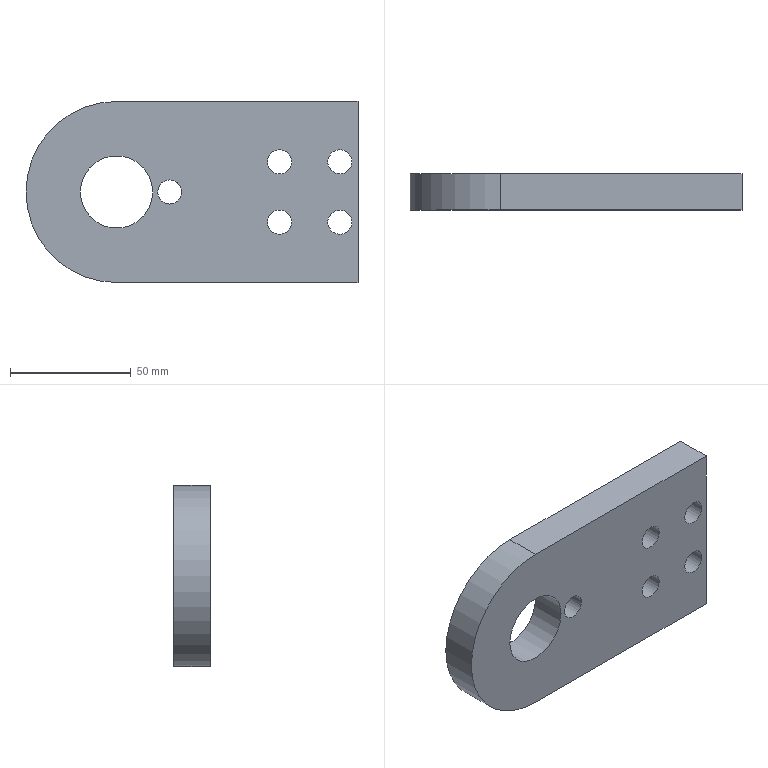Component | NX | DRILL_JIG_BUSH | 1 solid | 12 faces | box 137.5 x 15 x 75 mm | volume 129141 mm3 | cylinder 7 | plane 5 | commonest cylinder face diameters 10 x5 75 x1 30 x1
STEP:
#1=CARTESIAN_POINT('',(0.,0.,0.));
#2=DIRECTION('',(0.,0.,1.));
#3=DIRECTION('',(1.,0.,0.));
#4=AXIS2_PLACEMENT_3D('',#1,#2,#3);
#5=CARTESIAN_POINT('',(-28.675,85.796,25.));
#6=VERTEX_POINT('',#5);
#7=CARTESIAN_POINT('',(-28.675,85.796,100.));
#8=VERTEX_POINT('',#7);
#9=CARTESIAN_POINT('',(-28.675,85.796,62.5));
#10=DIRECTION('',(0.,1.,0.));
#11=DIRECTION('',(0.,0.,1.));
#12=AXIS2_PLACEMENT_3D('',#9,#10,#11);
#13=CIRCLE('',#12,37.5);
#14=CARTESIAN_POINT('',(-28.675,100.796,62.5));
#15=DIRECTION('',(0.,-1.,0.));
#16=DIRECTION('',(0.,0.,-1.));
#17=AXIS2_PLACEMENT_3D('',#14,#15,#16);
#18=CYLINDRICAL_SURFACE('',#17,37.5);
#19=CARTESIAN_POINT('',(9.425,15.));
#20=DIRECTION('',(-1.,0.));
#21=VECTOR('',#20,1.);
#22=LINE('',#19,#21);
#23=(GEOMETRIC_REPRESENTATION_CONTEXT(2)PARAMETRIC_REPRESENTATION_CONTEXT()REPRESENTATION_CONTEXT('',''));
#24=DEFINITIONAL_REPRESENTATION('',(#22),#23);
#25=PCURVE('',#18,#24);
#26=CARTESIAN_POINT('',(-28.675,85.796,62.5));
#27=DIRECTION('',(0.,1.,0.));
#28=DIRECTION('',(0.,0.,1.));
#29=AXIS2_PLACEMENT_3D('',#26,#27,#28);
#30=PLANE('',#29);
#31=CARTESIAN_POINT('',(0.,0.));
#32=DIRECTION('',(1.,0.));
#33=AXIS2_PLACEMENT_2D('',#31,#32);
#34=CIRCLE('',#33,37.5);
#35=(GEOMETRIC_REPRESENTATION_CONTEXT(2)PARAMETRIC_REPRESENTATION_CONTEXT()REPRESENTATION_CONTEXT('',''));
#36=DEFINITIONAL_REPRESENTATION('',(#34),#35);
#37=PCURVE('',#30,#36);
#38=SURFACE_CURVE('',#13,(#25,#37),.PCURVE_S1.);
#39=EDGE_CURVE('',#6,#8,#38,.T.);
#40=ORIENTED_EDGE('',*,*,#39,.T.);
#41=CARTESIAN_POINT('',(-28.675,100.796,100.));
#42=VERTEX_POINT('',#41);
#43=CARTESIAN_POINT('',(-28.675,93.296,100.));
#44=DIRECTION('',(0.,-1.,0.));
#45=VECTOR('',#44,1.);
#46=LINE('',#43,#45);
#47=CARTESIAN_POINT('',(3.142,7.5));
#48=DIRECTION('',(0.,1.));
#49=VECTOR('',#48,1.);
#50=LINE('',#47,#49);
#51=(GEOMETRIC_REPRESENTATION_CONTEXT(2)PARAMETRIC_REPRESENTATION_CONTEXT()REPRESENTATION_CONTEXT('',''));
#52=DEFINITIONAL_REPRESENTATION('',(#50),#51);
#53=PCURVE('',#18,#52);
#54=CARTESIAN_POINT('',(-28.675,100.796,100.));
#55=DIRECTION('',(0.,0.,-1.));
#56=DIRECTION('',(-1.,0.,0.));
#57=AXIS2_PLACEMENT_3D('',#54,#55,#56);
#58=PLANE('',#57);
#59=CARTESIAN_POINT('',(0.,-7.5));
#60=DIRECTION('',(0.,-1.));
#61=VECTOR('',#60,1.);
#62=LINE('',#59,#61);
#63=(GEOMETRIC_REPRESENTATION_CONTEXT(2)PARAMETRIC_REPRESENTATION_CONTEXT()REPRESENTATION_CONTEXT('',''));
#64=DEFINITIONAL_REPRESENTATION('',(#62),#63);
#65=PCURVE('',#58,#64);
#66=SURFACE_CURVE('',#46,(#53,#65),.PCURVE_S1.);
#67=EDGE_CURVE('',#42,#8,#66,.T.);
#68=ORIENTED_EDGE('',*,*,#67,.F.);
#69=CARTESIAN_POINT('',(-28.675,100.796,25.));
#70=VERTEX_POINT('',#69);
#71=CARTESIAN_POINT('',(-28.675,100.796,62.5));
#72=DIRECTION('',(0.,1.,0.));
#73=DIRECTION('',(0.,0.,1.));
#74=AXIS2_PLACEMENT_3D('',#71,#72,#73);
#75=CIRCLE('',#74,37.5);
#76=CARTESIAN_POINT('',(9.425,0.));
#77=DIRECTION('',(-1.,0.));
#78=VECTOR('',#77,1.);
#79=LINE('',#76,#78);
#80=(GEOMETRIC_REPRESENTATION_CONTEXT(2)PARAMETRIC_REPRESENTATION_CONTEXT()REPRESENTATION_CONTEXT('',''));
#81=DEFINITIONAL_REPRESENTATION('',(#79),#80);
#82=PCURVE('',#18,#81);
#83=CARTESIAN_POINT('',(-28.675,100.796,62.5));
#84=DIRECTION('',(0.,1.,0.));
#85=DIRECTION('',(0.,0.,1.));
#86=AXIS2_PLACEMENT_3D('',#83,#84,#85);
#87=PLANE('',#86);
#88=CARTESIAN_POINT('',(0.,0.));
#89=DIRECTION('',(1.,0.));
#90=AXIS2_PLACEMENT_2D('',#88,#89);
#91=CIRCLE('',#90,37.5);
#92=(GEOMETRIC_REPRESENTATION_CONTEXT(2)PARAMETRIC_REPRESENTATION_CONTEXT()REPRESENTATION_CONTEXT('',''));
#93=DEFINITIONAL_REPRESENTATION('',(#91),#92);
#94=PCURVE('',#87,#93);
#95=SURFACE_CURVE('',#75,(#82,#94),.PCURVE_S1.);
#96=EDGE_CURVE('',#70,#42,#95,.T.);
#97=ORIENTED_EDGE('',*,*,#96,.F.);
#98=CARTESIAN_POINT('',(-28.675,93.296,25.));
#99=DIRECTION('',(0.,-1.,0.));
#100=VECTOR('',#99,1.);
#101=LINE('',#98,#100);
#102=CARTESIAN_POINT('',(6.283,7.5));
#103=DIRECTION('',(0.,1.));
#104=VECTOR('',#103,1.);
#105=LINE('',#102,#104);
#106=(GEOMETRIC_REPRESENTATION_CONTEXT(2)PARAMETRIC_REPRESENTATION_CONTEXT()REPRESENTATION_CONTEXT('',''));
#107=DEFINITIONAL_REPRESENTATION('',(#105),#106);
#108=PCURVE('',#18,#107);
#109=CARTESIAN_POINT('',(71.325,100.796,25.));
#110=DIRECTION('',(0.,0.,1.));
#111=DIRECTION('',(1.,0.,0.));
#112=AXIS2_PLACEMENT_3D('',#109,#110,#111);
#113=PLANE('',#112);
#114=CARTESIAN_POINT('',(-100.,-7.5));
#115=DIRECTION('',(0.,-1.));
#116=VECTOR('',#115,1.);
#117=LINE('',#114,#116);
#118=(GEOMETRIC_REPRESENTATION_CONTEXT(2)PARAMETRIC_REPRESENTATION_CONTEXT()REPRESENTATION_CONTEXT('',''));
#119=DEFINITIONAL_REPRESENTATION('',(#117),#118);
#120=PCURVE('',#113,#119);
#121=SURFACE_CURVE('',#101,(#108,#120),.PCURVE_S1.);
#122=EDGE_CURVE('',#70,#6,#121,.T.);
#123=ORIENTED_EDGE('',*,*,#122,.T.);
#124=EDGE_LOOP('',(#40,#68,#97,#123));
#125=FACE_BOUND('',#124,.T.);
#126=ADVANCED_FACE('',(#125),#18,.T.);
#127=CARTESIAN_POINT('',(71.325,85.796,100.));
#128=VERTEX_POINT('',#127);
#129=CARTESIAN_POINT('',(-28.675,85.796,100.));
#130=DIRECTION('',(1.,0.,0.));
#131=VECTOR('',#130,1.);
#132=LINE('',#129,#131);
#133=CARTESIAN_POINT('',(0.,-15.));
#134=DIRECTION('',(-1.,0.));
#135=VECTOR('',#134,1.);
#136=LINE('',#133,#135);
#137=(GEOMETRIC_REPRESENTATION_CONTEXT(2)PARAMETRIC_REPRESENTATION_CONTEXT()REPRESENTATION_CONTEXT('',''));
#138=DEFINITIONAL_REPRESENTATION('',(#136),#137);
#139=PCURVE('',#58,#138);
#140=CARTESIAN_POINT('',(37.5,0.));
#141=DIRECTION('',(0.,1.));
#142=VECTOR('',#141,1.);
#143=LINE('',#140,#142);
#144=(GEOMETRIC_REPRESENTATION_CONTEXT(2)PARAMETRIC_REPRESENTATION_CONTEXT()REPRESENTATION_CONTEXT('',''));
#145=DEFINITIONAL_REPRESENTATION('',(#143),#144);
#146=PCURVE('',#30,#145);
#147=SURFACE_CURVE('',#132,(#139,#146),.PCURVE_S1.);
#148=EDGE_CURVE('',#8,#128,#147,.T.);
#149=ORIENTED_EDGE('',*,*,#148,.T.);
#150=CARTESIAN_POINT('',(71.325,100.796,100.));
#151=VERTEX_POINT('',#150);
#152=CARTESIAN_POINT('',(71.325,100.796,100.));
#153=DIRECTION('',(0.,-1.,0.));
#154=VECTOR('',#153,1.);
#155=LINE('',#152,#154);
#156=CARTESIAN_POINT('',(-100.,0.));
#157=DIRECTION('',(0.,-1.));
#158=VECTOR('',#157,1.);
#159=LINE('',#156,#158);
#160=(GEOMETRIC_REPRESENTATION_CONTEXT(2)PARAMETRIC_REPRESENTATION_CONTEXT()REPRESENTATION_CONTEXT('',''));
#161=DEFINITIONAL_REPRESENTATION('',(#159),#160);
#162=PCURVE('',#58,#161);
#163=CARTESIAN_POINT('',(71.325,100.796,112.5));
#164=DIRECTION('',(-1.,0.,-0.));
#165=DIRECTION('',(-0.,0.,1.));
#166=AXIS2_PLACEMENT_3D('',#163,#164,#165);
#167=PLANE('',#166);
#168=CARTESIAN_POINT('',(-12.5,0.));
#169=DIRECTION('',(0.,-1.));
#170=VECTOR('',#169,1.);
#171=LINE('',#168,#170);
#172=(GEOMETRIC_REPRESENTATION_CONTEXT(2)PARAMETRIC_REPRESENTATION_CONTEXT()REPRESENTATION_CONTEXT('',''));
#173=DEFINITIONAL_REPRESENTATION('',(#171),#172);
#174=PCURVE('',#167,#173);
#175=SURFACE_CURVE('',#155,(#162,#174),.PCURVE_S1.);
#176=EDGE_CURVE('',#151,#128,#175,.T.);
#177=ORIENTED_EDGE('',*,*,#176,.F.);
#178=CARTESIAN_POINT('',(-28.675,100.796,100.));
#179=DIRECTION('',(1.,0.,0.));
#180=VECTOR('',#179,1.);
#181=LINE('',#178,#180);
#182=CARTESIAN_POINT('',(0.,0.));
#183=DIRECTION('',(-1.,0.));
#184=VECTOR('',#183,1.);
#185=LINE('',#182,#184);
#186=(GEOMETRIC_REPRESENTATION_CONTEXT(2)PARAMETRIC_REPRESENTATION_CONTEXT()REPRESENTATION_CONTEXT('',''));
#187=DEFINITIONAL_REPRESENTATION('',(#185),#186);
#188=PCURVE('',#58,#187);
#189=CARTESIAN_POINT('',(37.5,0.));
#190=DIRECTION('',(0.,1.));
#191=VECTOR('',#190,1.);
#192=LINE('',#189,#191);
#193=(GEOMETRIC_REPRESENTATION_CONTEXT(2)PARAMETRIC_REPRESENTATION_CONTEXT()REPRESENTATION_CONTEXT('',''));
#194=DEFINITIONAL_REPRESENTATION('',(#192),#193);
#195=PCURVE('',#87,#194);
#196=SURFACE_CURVE('',#181,(#188,#195),.PCURVE_S1.);
#197=EDGE_CURVE('',#42,#151,#196,.T.);
#198=ORIENTED_EDGE('',*,*,#197,.F.);
#199=ORIENTED_EDGE('',*,*,#67,.T.);
#200=EDGE_LOOP('',(#149,#177,#198,#199));
#201=FACE_BOUND('',#200,.T.);
#202=ADVANCED_FACE('',(#201),#58,.F.);
#203=CARTESIAN_POINT('',(71.325,85.796,25.));
#204=VERTEX_POINT('',#203);
#205=CARTESIAN_POINT('',(71.325,85.796,112.5));
#206=DIRECTION('',(0.,0.,-1.));
#207=VECTOR('',#206,1.);
#208=LINE('',#205,#207);
#209=CARTESIAN_POINT('',(0.,-15.));
#210=DIRECTION('',(-1.,0.));
#211=VECTOR('',#210,1.);
#212=LINE('',#209,#211);
#213=(GEOMETRIC_REPRESENTATION_CONTEXT(2)PARAMETRIC_REPRESENTATION_CONTEXT()REPRESENTATION_CONTEXT('',''));
#214=DEFINITIONAL_REPRESENTATION('',(#212),#213);
#215=PCURVE('',#167,#214);
#216=CARTESIAN_POINT('',(50.,100.));
#217=DIRECTION('',(-1.,0.));
#218=VECTOR('',#217,1.);
#219=LINE('',#216,#218);
#220=(GEOMETRIC_REPRESENTATION_CONTEXT(2)PARAMETRIC_REPRESENTATION_CONTEXT()REPRESENTATION_CONTEXT('',''));
#221=DEFINITIONAL_REPRESENTATION('',(#219),#220);
#222=PCURVE('',#30,#221);
#223=SURFACE_CURVE('',#208,(#215,#222),.PCURVE_S1.);
#224=EDGE_CURVE('',#128,#204,#223,.T.);
#225=ORIENTED_EDGE('',*,*,#224,.T.);
#226=CARTESIAN_POINT('',(71.325,100.796,25.));
#227=VERTEX_POINT('',#226);
#228=CARTESIAN_POINT('',(71.325,100.796,25.));
#229=DIRECTION('',(0.,-1.,0.));
#230=VECTOR('',#229,1.);
#231=LINE('',#228,#230);
#232=CARTESIAN_POINT('',(-87.5,0.));
#233=DIRECTION('',(0.,-1.));
#234=VECTOR('',#233,1.);
#235=LINE('',#232,#234);
#236=(GEOMETRIC_REPRESENTATION_CONTEXT(2)PARAMETRIC_REPRESENTATION_CONTEXT()REPRESENTATION_CONTEXT('',''));
#237=DEFINITIONAL_REPRESENTATION('',(#235),#236);
#238=PCURVE('',#167,#237);
#239=CARTESIAN_POINT('',(0.,0.));
#240=DIRECTION('',(0.,-1.));
#241=VECTOR('',#240,1.);
#242=LINE('',#239,#241);
#243=(GEOMETRIC_REPRESENTATION_CONTEXT(2)PARAMETRIC_REPRESENTATION_CONTEXT()REPRESENTATION_CONTEXT('',''));
#244=DEFINITIONAL_REPRESENTATION('',(#242),#243);
#245=PCURVE('',#113,#244);
#246=SURFACE_CURVE('',#231,(#238,#245),.PCURVE_S1.);
#247=EDGE_CURVE('',#227,#204,#246,.T.);
#248=ORIENTED_EDGE('',*,*,#247,.F.);
#249=CARTESIAN_POINT('',(71.325,100.796,112.5));
#250=DIRECTION('',(0.,0.,-1.));
#251=VECTOR('',#250,1.);
#252=LINE('',#249,#251);
#253=CARTESIAN_POINT('',(0.,0.));
#254=DIRECTION('',(-1.,0.));
#255=VECTOR('',#254,1.);
#256=LINE('',#253,#255);
#257=(GEOMETRIC_REPRESENTATION_CONTEXT(2)PARAMETRIC_REPRESENTATION_CONTEXT()REPRESENTATION_CONTEXT('',''));
#258=DEFINITIONAL_REPRESENTATION('',(#256),#257);
#259=PCURVE('',#167,#258);
#260=CARTESIAN_POINT('',(50.,100.));
#261=DIRECTION('',(-1.,0.));
#262=VECTOR('',#261,1.);
#263=LINE('',#260,#262);
#264=(GEOMETRIC_REPRESENTATION_CONTEXT(2)PARAMETRIC_REPRESENTATION_CONTEXT()REPRESENTATION_CONTEXT('',''));
#265=DEFINITIONAL_REPRESENTATION('',(#263),#264);
#266=PCURVE('',#87,#265);
#267=SURFACE_CURVE('',#252,(#259,#266),.PCURVE_S1.);
#268=EDGE_CURVE('',#151,#227,#267,.T.);
#269=ORIENTED_EDGE('',*,*,#268,.F.);
#270=ORIENTED_EDGE('',*,*,#176,.T.);
#271=EDGE_LOOP('',(#225,#248,#269,#270));
#272=FACE_BOUND('',#271,.T.);
#273=ADVANCED_FACE('',(#272),#167,.F.);
#274=CARTESIAN_POINT('',(58.825,100.796,50.));
#275=VERTEX_POINT('',#274);
#276=CARTESIAN_POINT('',(63.825,100.796,50.));
#277=DIRECTION('',(0.,1.,0.));
#278=DIRECTION('',(-1.,0.,0.));
#279=AXIS2_PLACEMENT_3D('',#276,#277,#278);
#280=CIRCLE('',#279,5.);
#281=CARTESIAN_POINT('',(63.825,100.796,50.));
#282=DIRECTION('',(0.,-1.,0.));
#283=DIRECTION('',(0.,0.,-1.));
#284=AXIS2_PLACEMENT_3D('',#281,#282,#283);
#285=CYLINDRICAL_SURFACE('',#284,5.);
#286=CARTESIAN_POINT('',(10.996,0.));
#287=DIRECTION('',(-1.,0.));
#288=VECTOR('',#287,1.);
#289=LINE('',#286,#288);
#290=(GEOMETRIC_REPRESENTATION_CONTEXT(2)PARAMETRIC_REPRESENTATION_CONTEXT()REPRESENTATION_CONTEXT('',''));
#291=DEFINITIONAL_REPRESENTATION('',(#289),#290);
#292=PCURVE('',#285,#291);
#293=CARTESIAN_POINT('',(-12.5,92.5));
#294=DIRECTION('',(0.,-1.));
#295=AXIS2_PLACEMENT_2D('',#293,#294);
#296=CIRCLE('',#295,5.);
#297=(GEOMETRIC_REPRESENTATION_CONTEXT(2)PARAMETRIC_REPRESENTATION_CONTEXT()REPRESENTATION_CONTEXT('',''));
#298=DEFINITIONAL_REPRESENTATION('',(#296),#297);
#299=PCURVE('',#87,#298);
#300=SURFACE_CURVE('',#280,(#292,#299),.PCURVE_S1.);
#301=EDGE_CURVE('',#275,#275,#300,.T.);
#302=ORIENTED_EDGE('',*,*,#301,.F.);
#303=CARTESIAN_POINT('',(58.825,85.796,50.));
#304=VERTEX_POINT('',#303);
#305=CARTESIAN_POINT('',(58.825,100.796,50.));
#306=CARTESIAN_POINT('',(58.825,85.796,50.));
#307=B_SPLINE_CURVE_WITH_KNOTS('',1,(#305,#306),.UNSPECIFIED.,.F.,.F.,(2,2),(0.,15.),.PIECEWISE_BEZIER_KNOTS.);
#308=CARTESIAN_POINT('',(10.996,0.));
#309=DIRECTION('',(0.,1.));
#310=VECTOR('',#309,1.);
#311=LINE('',#308,#310);
#312=(GEOMETRIC_REPRESENTATION_CONTEXT(2)PARAMETRIC_REPRESENTATION_CONTEXT()REPRESENTATION_CONTEXT('',''));
#313=DEFINITIONAL_REPRESENTATION('',(#311),#312);
#314=PCURVE('',#285,#313);
#315=CARTESIAN_POINT('',(4.712,0.));
#316=DIRECTION('',(0.,1.));
#317=VECTOR('',#316,1.);
#318=LINE('',#315,#317);
#319=(GEOMETRIC_REPRESENTATION_CONTEXT(2)PARAMETRIC_REPRESENTATION_CONTEXT()REPRESENTATION_CONTEXT('',''));
#320=DEFINITIONAL_REPRESENTATION('',(#318),#319);
#321=PCURVE('',#285,#320);
#322=SEAM_CURVE('',#307,(#314,#321),.PCURVE_S1.);
#323=EDGE_CURVE('',#275,#304,#322,.T.);
#324=ORIENTED_EDGE('',*,*,#323,.T.);
#325=CARTESIAN_POINT('',(63.825,85.796,50.));
#326=DIRECTION('',(0.,1.,0.));
#327=DIRECTION('',(-1.,0.,0.));
#328=AXIS2_PLACEMENT_3D('',#325,#326,#327);
#329=CIRCLE('',#328,5.);
#330=CARTESIAN_POINT('',(10.996,15.));
#331=DIRECTION('',(-1.,0.));
#332=VECTOR('',#331,1.);
#333=LINE('',#330,#332);
#334=(GEOMETRIC_REPRESENTATION_CONTEXT(2)PARAMETRIC_REPRESENTATION_CONTEXT()REPRESENTATION_CONTEXT('',''));
#335=DEFINITIONAL_REPRESENTATION('',(#333),#334);
#336=PCURVE('',#285,#335);
#337=CARTESIAN_POINT('',(-12.5,92.5));
#338=DIRECTION('',(0.,-1.));
#339=AXIS2_PLACEMENT_2D('',#337,#338);
#340=CIRCLE('',#339,5.);
#341=(GEOMETRIC_REPRESENTATION_CONTEXT(2)PARAMETRIC_REPRESENTATION_CONTEXT()REPRESENTATION_CONTEXT('',''));
#342=DEFINITIONAL_REPRESENTATION('',(#340),#341);
#343=PCURVE('',#30,#342);
#344=SURFACE_CURVE('',#329,(#336,#343),.PCURVE_S1.);
#345=EDGE_CURVE('',#304,#304,#344,.T.);
#346=ORIENTED_EDGE('',*,*,#345,.T.);
#347=ORIENTED_EDGE('',*,*,#323,.F.);
#348=EDGE_LOOP('',(#302,#324,#346,#347));
#349=FACE_BOUND('',#348,.F.);
#350=ADVANCED_FACE('',(#349),#285,.F.);
#351=CARTESIAN_POINT('',(33.825,100.796,75.));
#352=VERTEX_POINT('',#351);
#353=CARTESIAN_POINT('',(38.825,100.796,75.));
#354=DIRECTION('',(0.,1.,0.));
#355=DIRECTION('',(-1.,0.,0.));
#356=AXIS2_PLACEMENT_3D('',#353,#354,#355);
#357=CIRCLE('',#356,5.);
#358=CARTESIAN_POINT('',(38.825,100.796,75.));
#359=DIRECTION('',(0.,-1.,0.));
#360=DIRECTION('',(0.,0.,-1.));
#361=AXIS2_PLACEMENT_3D('',#358,#359,#360);
#362=CYLINDRICAL_SURFACE('',#361,5.);
#363=CARTESIAN_POINT('',(10.996,0.));
#364=DIRECTION('',(-1.,0.));
#365=VECTOR('',#364,1.);
#366=LINE('',#363,#365);
#367=(GEOMETRIC_REPRESENTATION_CONTEXT(2)PARAMETRIC_REPRESENTATION_CONTEXT()REPRESENTATION_CONTEXT('',''));
#368=DEFINITIONAL_REPRESENTATION('',(#366),#367);
#369=PCURVE('',#362,#368);
#370=CARTESIAN_POINT('',(12.5,67.5));
#371=DIRECTION('',(0.,-1.));
#372=AXIS2_PLACEMENT_2D('',#370,#371);
#373=CIRCLE('',#372,5.);
#374=(GEOMETRIC_REPRESENTATION_CONTEXT(2)PARAMETRIC_REPRESENTATION_CONTEXT()REPRESENTATION_CONTEXT('',''));
#375=DEFINITIONAL_REPRESENTATION('',(#373),#374);
#376=PCURVE('',#87,#375);
#377=SURFACE_CURVE('',#357,(#369,#376),.PCURVE_S1.);
#378=EDGE_CURVE('',#352,#352,#377,.T.);
#379=ORIENTED_EDGE('',*,*,#378,.F.);
#380=CARTESIAN_POINT('',(33.825,85.796,75.));
#381=VERTEX_POINT('',#380);
#382=CARTESIAN_POINT('',(33.825,100.796,75.));
#383=CARTESIAN_POINT('',(33.825,85.796,75.));
#384=B_SPLINE_CURVE_WITH_KNOTS('',1,(#382,#383),.UNSPECIFIED.,.F.,.F.,(2,2),(0.,15.),.PIECEWISE_BEZIER_KNOTS.);
#385=CARTESIAN_POINT('',(10.996,0.));
#386=DIRECTION('',(0.,1.));
#387=VECTOR('',#386,1.);
#388=LINE('',#385,#387);
#389=(GEOMETRIC_REPRESENTATION_CONTEXT(2)PARAMETRIC_REPRESENTATION_CONTEXT()REPRESENTATION_CONTEXT('',''));
#390=DEFINITIONAL_REPRESENTATION('',(#388),#389);
#391=PCURVE('',#362,#390);
#392=CARTESIAN_POINT('',(4.712,0.));
#393=DIRECTION('',(0.,1.));
#394=VECTOR('',#393,1.);
#395=LINE('',#392,#394);
#396=(GEOMETRIC_REPRESENTATION_CONTEXT(2)PARAMETRIC_REPRESENTATION_CONTEXT()REPRESENTATION_CONTEXT('',''));
#397=DEFINITIONAL_REPRESENTATION('',(#395),#396);
#398=PCURVE('',#362,#397);
#399=SEAM_CURVE('',#384,(#391,#398),.PCURVE_S1.);
#400=EDGE_CURVE('',#352,#381,#399,.T.);
#401=ORIENTED_EDGE('',*,*,#400,.T.);
#402=CARTESIAN_POINT('',(38.825,85.796,75.));
#403=DIRECTION('',(0.,1.,0.));
#404=DIRECTION('',(-1.,0.,0.));
#405=AXIS2_PLACEMENT_3D('',#402,#403,#404);
#406=CIRCLE('',#405,5.);
#407=CARTESIAN_POINT('',(10.996,15.));
#408=DIRECTION('',(-1.,0.));
#409=VECTOR('',#408,1.);
#410=LINE('',#407,#409);
#411=(GEOMETRIC_REPRESENTATION_CONTEXT(2)PARAMETRIC_REPRESENTATION_CONTEXT()REPRESENTATION_CONTEXT('',''));
#412=DEFINITIONAL_REPRESENTATION('',(#410),#411);
#413=PCURVE('',#362,#412);
#414=CARTESIAN_POINT('',(12.5,67.5));
#415=DIRECTION('',(0.,-1.));
#416=AXIS2_PLACEMENT_2D('',#414,#415);
#417=CIRCLE('',#416,5.);
#418=(GEOMETRIC_REPRESENTATION_CONTEXT(2)PARAMETRIC_REPRESENTATION_CONTEXT()REPRESENTATION_CONTEXT('',''));
#419=DEFINITIONAL_REPRESENTATION('',(#417),#418);
#420=PCURVE('',#30,#419);
#421=SURFACE_CURVE('',#406,(#413,#420),.PCURVE_S1.);
#422=EDGE_CURVE('',#381,#381,#421,.T.);
#423=ORIENTED_EDGE('',*,*,#422,.T.);
#424=ORIENTED_EDGE('',*,*,#400,.F.);
#425=EDGE_LOOP('',(#379,#401,#423,#424));
#426=FACE_BOUND('',#425,.F.);
#427=ADVANCED_FACE('',(#426),#362,.F.);
#428=CARTESIAN_POINT('',(33.825,100.796,50.));
#429=VERTEX_POINT('',#428);
#430=CARTESIAN_POINT('',(38.825,100.796,50.));
#431=DIRECTION('',(0.,1.,0.));
#432=DIRECTION('',(-1.,0.,0.));
#433=AXIS2_PLACEMENT_3D('',#430,#431,#432);
#434=CIRCLE('',#433,5.);
#435=CARTESIAN_POINT('',(38.825,100.796,50.));
#436=DIRECTION('',(0.,-1.,0.));
#437=DIRECTION('',(0.,0.,-1.));
#438=AXIS2_PLACEMENT_3D('',#435,#436,#437);
#439=CYLINDRICAL_SURFACE('',#438,5.);
#440=CARTESIAN_POINT('',(10.996,0.));
#441=DIRECTION('',(-1.,0.));
#442=VECTOR('',#441,1.);
#443=LINE('',#440,#442);
#444=(GEOMETRIC_REPRESENTATION_CONTEXT(2)PARAMETRIC_REPRESENTATION_CONTEXT()REPRESENTATION_CONTEXT('',''));
#445=DEFINITIONAL_REPRESENTATION('',(#443),#444);
#446=PCURVE('',#439,#445);
#447=CARTESIAN_POINT('',(-12.5,67.5));
#448=DIRECTION('',(0.,-1.));
#449=AXIS2_PLACEMENT_2D('',#447,#448);
#450=CIRCLE('',#449,5.);
#451=(GEOMETRIC_REPRESENTATION_CONTEXT(2)PARAMETRIC_REPRESENTATION_CONTEXT()REPRESENTATION_CONTEXT('',''));
#452=DEFINITIONAL_REPRESENTATION('',(#450),#451);
#453=PCURVE('',#87,#452);
#454=SURFACE_CURVE('',#434,(#446,#453),.PCURVE_S1.);
#455=EDGE_CURVE('',#429,#429,#454,.T.);
#456=ORIENTED_EDGE('',*,*,#455,.F.);
#457=CARTESIAN_POINT('',(33.825,85.796,50.));
#458=VERTEX_POINT('',#457);
#459=CARTESIAN_POINT('',(33.825,100.796,50.));
#460=CARTESIAN_POINT('',(33.825,85.796,50.));
#461=B_SPLINE_CURVE_WITH_KNOTS('',1,(#459,#460),.UNSPECIFIED.,.F.,.F.,(2,2),(0.,15.),.PIECEWISE_BEZIER_KNOTS.);
#462=CARTESIAN_POINT('',(10.996,0.));
#463=DIRECTION('',(0.,1.));
#464=VECTOR('',#463,1.);
#465=LINE('',#462,#464);
#466=(GEOMETRIC_REPRESENTATION_CONTEXT(2)PARAMETRIC_REPRESENTATION_CONTEXT()REPRESENTATION_CONTEXT('',''));
#467=DEFINITIONAL_REPRESENTATION('',(#465),#466);
#468=PCURVE('',#439,#467);
#469=CARTESIAN_POINT('',(4.712,0.));
#470=DIRECTION('',(0.,1.));
#471=VECTOR('',#470,1.);
#472=LINE('',#469,#471);
#473=(GEOMETRIC_REPRESENTATION_CONTEXT(2)PARAMETRIC_REPRESENTATION_CONTEXT()REPRESENTATION_CONTEXT('',''));
#474=DEFINITIONAL_REPRESENTATION('',(#472),#473);
#475=PCURVE('',#439,#474);
#476=SEAM_CURVE('',#461,(#468,#475),.PCURVE_S1.);
#477=EDGE_CURVE('',#429,#458,#476,.T.);
#478=ORIENTED_EDGE('',*,*,#477,.T.);
#479=CARTESIAN_POINT('',(38.825,85.796,50.));
#480=DIRECTION('',(0.,1.,0.));
#481=DIRECTION('',(-1.,0.,0.));
#482=AXIS2_PLACEMENT_3D('',#479,#480,#481);
#483=CIRCLE('',#482,5.);
#484=CARTESIAN_POINT('',(10.996,15.));
#485=DIRECTION('',(-1.,0.));
#486=VECTOR('',#485,1.);
#487=LINE('',#484,#486);
#488=(GEOMETRIC_REPRESENTATION_CONTEXT(2)PARAMETRIC_REPRESENTATION_CONTEXT()REPRESENTATION_CONTEXT('',''));
#489=DEFINITIONAL_REPRESENTATION('',(#487),#488);
#490=PCURVE('',#439,#489);
#491=CARTESIAN_POINT('',(-12.5,67.5));
#492=DIRECTION('',(0.,-1.));
#493=AXIS2_PLACEMENT_2D('',#491,#492);
#494=CIRCLE('',#493,5.);
#495=(GEOMETRIC_REPRESENTATION_CONTEXT(2)PARAMETRIC_REPRESENTATION_CONTEXT()REPRESENTATION_CONTEXT('',''));
#496=DEFINITIONAL_REPRESENTATION('',(#494),#495);
#497=PCURVE('',#30,#496);
#498=SURFACE_CURVE('',#483,(#490,#497),.PCURVE_S1.);
#499=EDGE_CURVE('',#458,#458,#498,.T.);
#500=ORIENTED_EDGE('',*,*,#499,.T.);
#501=ORIENTED_EDGE('',*,*,#477,.F.);
#502=EDGE_LOOP('',(#456,#478,#500,#501));
#503=FACE_BOUND('',#502,.F.);
#504=ADVANCED_FACE('',(#503),#439,.F.);
#505=CARTESIAN_POINT('',(-43.675,100.796,62.5));
#506=VERTEX_POINT('',#505);
#507=CARTESIAN_POINT('',(-28.675,100.796,62.5));
#508=DIRECTION('',(0.,1.,0.));
#509=DIRECTION('',(-1.,0.,0.));
#510=AXIS2_PLACEMENT_3D('',#507,#508,#509);
#511=CIRCLE('',#510,15.);
#512=CARTESIAN_POINT('',(-28.675,100.796,62.5));
#513=DIRECTION('',(0.,-1.,0.));
#514=DIRECTION('',(0.,0.,-1.));
#515=AXIS2_PLACEMENT_3D('',#512,#513,#514);
#516=CYLINDRICAL_SURFACE('',#515,15.);
#517=CARTESIAN_POINT('',(10.996,0.));
#518=DIRECTION('',(-1.,0.));
#519=VECTOR('',#518,1.);
#520=LINE('',#517,#519);
#521=(GEOMETRIC_REPRESENTATION_CONTEXT(2)PARAMETRIC_REPRESENTATION_CONTEXT()REPRESENTATION_CONTEXT('',''));
#522=DEFINITIONAL_REPRESENTATION('',(#520),#521);
#523=PCURVE('',#516,#522);
#524=CARTESIAN_POINT('',(0.,0.));
#525=DIRECTION('',(0.,-1.));
#526=AXIS2_PLACEMENT_2D('',#524,#525);
#527=CIRCLE('',#526,15.);
#528=(GEOMETRIC_REPRESENTATION_CONTEXT(2)PARAMETRIC_REPRESENTATION_CONTEXT()REPRESENTATION_CONTEXT('',''));
#529=DEFINITIONAL_REPRESENTATION('',(#527),#528);
#530=PCURVE('',#87,#529);
#531=SURFACE_CURVE('',#511,(#523,#530),.PCURVE_S1.);
#532=EDGE_CURVE('',#506,#506,#531,.T.);
#533=ORIENTED_EDGE('',*,*,#532,.F.);
#534=CARTESIAN_POINT('',(-43.675,85.796,62.5));
#535=VERTEX_POINT('',#534);
#536=CARTESIAN_POINT('',(-43.675,100.796,62.5));
#537=CARTESIAN_POINT('',(-43.675,85.796,62.5));
#538=B_SPLINE_CURVE_WITH_KNOTS('',1,(#536,#537),.UNSPECIFIED.,.F.,.F.,(2,2),(0.,15.),.PIECEWISE_BEZIER_KNOTS.);
#539=CARTESIAN_POINT('',(10.996,0.));
#540=DIRECTION('',(0.,1.));
#541=VECTOR('',#540,1.);
#542=LINE('',#539,#541);
#543=(GEOMETRIC_REPRESENTATION_CONTEXT(2)PARAMETRIC_REPRESENTATION_CONTEXT()REPRESENTATION_CONTEXT('',''));
#544=DEFINITIONAL_REPRESENTATION('',(#542),#543);
#545=PCURVE('',#516,#544);
#546=CARTESIAN_POINT('',(4.712,0.));
#547=DIRECTION('',(0.,1.));
#548=VECTOR('',#547,1.);
#549=LINE('',#546,#548);
#550=(GEOMETRIC_REPRESENTATION_CONTEXT(2)PARAMETRIC_REPRESENTATION_CONTEXT()REPRESENTATION_CONTEXT('',''));
#551=DEFINITIONAL_REPRESENTATION('',(#549),#550);
#552=PCURVE('',#516,#551);
#553=SEAM_CURVE('',#538,(#545,#552),.PCURVE_S1.);
#554=EDGE_CURVE('',#506,#535,#553,.T.);
#555=ORIENTED_EDGE('',*,*,#554,.T.);
#556=CARTESIAN_POINT('',(-28.675,85.796,62.5));
#557=DIRECTION('',(0.,1.,0.));
#558=DIRECTION('',(-1.,0.,0.));
#559=AXIS2_PLACEMENT_3D('',#556,#557,#558);
#560=CIRCLE('',#559,15.);
#561=CARTESIAN_POINT('',(10.996,15.));
#562=DIRECTION('',(-1.,0.));
#563=VECTOR('',#562,1.);
#564=LINE('',#561,#563);
#565=(GEOMETRIC_REPRESENTATION_CONTEXT(2)PARAMETRIC_REPRESENTATION_CONTEXT()REPRESENTATION_CONTEXT('',''));
#566=DEFINITIONAL_REPRESENTATION('',(#564),#565);
#567=PCURVE('',#516,#566);
#568=CARTESIAN_POINT('',(0.,0.));
#569=DIRECTION('',(0.,-1.));
#570=AXIS2_PLACEMENT_2D('',#568,#569);
#571=CIRCLE('',#570,15.);
#572=(GEOMETRIC_REPRESENTATION_CONTEXT(2)PARAMETRIC_REPRESENTATION_CONTEXT()REPRESENTATION_CONTEXT('',''));
#573=DEFINITIONAL_REPRESENTATION('',(#571),#572);
#574=PCURVE('',#30,#573);
#575=SURFACE_CURVE('',#560,(#567,#574),.PCURVE_S1.);
#576=EDGE_CURVE('',#535,#535,#575,.T.);
#577=ORIENTED_EDGE('',*,*,#576,.T.);
#578=ORIENTED_EDGE('',*,*,#554,.F.);
#579=EDGE_LOOP('',(#533,#555,#577,#578));
#580=FACE_BOUND('',#579,.F.);
#581=ADVANCED_FACE('',(#580),#516,.F.);
#582=CARTESIAN_POINT('',(71.325,85.796,25.));
#583=DIRECTION('',(-1.,0.,0.));
#584=VECTOR('',#583,1.);
#585=LINE('',#582,#584);
#586=CARTESIAN_POINT('',(0.,-15.));
#587=DIRECTION('',(-1.,0.));
#588=VECTOR('',#587,1.);
#589=LINE('',#586,#588);
#590=(GEOMETRIC_REPRESENTATION_CONTEXT(2)PARAMETRIC_REPRESENTATION_CONTEXT()REPRESENTATION_CONTEXT('',''));
#591=DEFINITIONAL_REPRESENTATION('',(#589),#590);
#592=PCURVE('',#113,#591);
#593=CARTESIAN_POINT('',(-37.5,100.));
#594=DIRECTION('',(0.,-1.));
#595=VECTOR('',#594,1.);
#596=LINE('',#593,#595);
#597=(GEOMETRIC_REPRESENTATION_CONTEXT(2)PARAMETRIC_REPRESENTATION_CONTEXT()REPRESENTATION_CONTEXT('',''));
#598=DEFINITIONAL_REPRESENTATION('',(#596),#597);
#599=PCURVE('',#30,#598);
#600=SURFACE_CURVE('',#585,(#592,#599),.PCURVE_S1.);
#601=EDGE_CURVE('',#204,#6,#600,.T.);
#602=ORIENTED_EDGE('',*,*,#601,.T.);
#603=ORIENTED_EDGE('',*,*,#122,.F.);
#604=CARTESIAN_POINT('',(71.325,100.796,25.));
#605=DIRECTION('',(-1.,0.,0.));
#606=VECTOR('',#605,1.);
#607=LINE('',#604,#606);
#608=CARTESIAN_POINT('',(0.,0.));
#609=DIRECTION('',(-1.,0.));
#610=VECTOR('',#609,1.);
#611=LINE('',#608,#610);
#612=(GEOMETRIC_REPRESENTATION_CONTEXT(2)PARAMETRIC_REPRESENTATION_CONTEXT()REPRESENTATION_CONTEXT('',''));
#613=DEFINITIONAL_REPRESENTATION('',(#611),#612);
#614=PCURVE('',#113,#613);
#615=CARTESIAN_POINT('',(-37.5,100.));
#616=DIRECTION('',(0.,-1.));
#617=VECTOR('',#616,1.);
#618=LINE('',#615,#617);
#619=(GEOMETRIC_REPRESENTATION_CONTEXT(2)PARAMETRIC_REPRESENTATION_CONTEXT()REPRESENTATION_CONTEXT('',''));
#620=DEFINITIONAL_REPRESENTATION('',(#618),#619);
#621=PCURVE('',#87,#620);
#622=SURFACE_CURVE('',#607,(#614,#621),.PCURVE_S1.);
#623=EDGE_CURVE('',#227,#70,#622,.T.);
#624=ORIENTED_EDGE('',*,*,#623,.F.);
#625=ORIENTED_EDGE('',*,*,#247,.T.);
#626=EDGE_LOOP('',(#602,#603,#624,#625));
#627=FACE_BOUND('',#626,.T.);
#628=ADVANCED_FACE('',(#627),#113,.F.);
#629=CARTESIAN_POINT('',(58.825,100.796,75.));
#630=VERTEX_POINT('',#629);
#631=CARTESIAN_POINT('',(63.825,100.796,75.));
#632=DIRECTION('',(0.,1.,0.));
#633=DIRECTION('',(-1.,0.,0.));
#634=AXIS2_PLACEMENT_3D('',#631,#632,#633);
#635=CIRCLE('',#634,5.);
#636=CARTESIAN_POINT('',(63.825,100.796,75.));
#637=DIRECTION('',(0.,-1.,0.));
#638=DIRECTION('',(0.,0.,-1.));
#639=AXIS2_PLACEMENT_3D('',#636,#637,#638);
#640=CYLINDRICAL_SURFACE('',#639,5.);
#641=CARTESIAN_POINT('',(10.996,0.));
#642=DIRECTION('',(-1.,0.));
#643=VECTOR('',#642,1.);
#644=LINE('',#641,#643);
#645=(GEOMETRIC_REPRESENTATION_CONTEXT(2)PARAMETRIC_REPRESENTATION_CONTEXT()REPRESENTATION_CONTEXT('',''));
#646=DEFINITIONAL_REPRESENTATION('',(#644),#645);
#647=PCURVE('',#640,#646);
#648=CARTESIAN_POINT('',(12.5,92.5));
#649=DIRECTION('',(0.,-1.));
#650=AXIS2_PLACEMENT_2D('',#648,#649);
#651=CIRCLE('',#650,5.);
#652=(GEOMETRIC_REPRESENTATION_CONTEXT(2)PARAMETRIC_REPRESENTATION_CONTEXT()REPRESENTATION_CONTEXT('',''));
#653=DEFINITIONAL_REPRESENTATION('',(#651),#652);
#654=PCURVE('',#87,#653);
#655=SURFACE_CURVE('',#635,(#647,#654),.PCURVE_S1.);
#656=EDGE_CURVE('',#630,#630,#655,.T.);
#657=ORIENTED_EDGE('',*,*,#656,.F.);
#658=CARTESIAN_POINT('',(58.825,85.796,75.));
#659=VERTEX_POINT('',#658);
#660=CARTESIAN_POINT('',(58.825,100.796,75.));
#661=CARTESIAN_POINT('',(58.825,85.796,75.));
#662=B_SPLINE_CURVE_WITH_KNOTS('',1,(#660,#661),.UNSPECIFIED.,.F.,.F.,(2,2),(0.,15.),.PIECEWISE_BEZIER_KNOTS.);
#663=CARTESIAN_POINT('',(10.996,0.));
#664=DIRECTION('',(0.,1.));
#665=VECTOR('',#664,1.);
#666=LINE('',#663,#665);
#667=(GEOMETRIC_REPRESENTATION_CONTEXT(2)PARAMETRIC_REPRESENTATION_CONTEXT()REPRESENTATION_CONTEXT('',''));
#668=DEFINITIONAL_REPRESENTATION('',(#666),#667);
#669=PCURVE('',#640,#668);
#670=CARTESIAN_POINT('',(4.712,0.));
#671=DIRECTION('',(0.,1.));
#672=VECTOR('',#671,1.);
#673=LINE('',#670,#672);
#674=(GEOMETRIC_REPRESENTATION_CONTEXT(2)PARAMETRIC_REPRESENTATION_CONTEXT()REPRESENTATION_CONTEXT('',''));
#675=DEFINITIONAL_REPRESENTATION('',(#673),#674);
#676=PCURVE('',#640,#675);
#677=SEAM_CURVE('',#662,(#669,#676),.PCURVE_S1.);
#678=EDGE_CURVE('',#630,#659,#677,.T.);
#679=ORIENTED_EDGE('',*,*,#678,.T.);
#680=CARTESIAN_POINT('',(63.825,85.796,75.));
#681=DIRECTION('',(0.,1.,0.));
#682=DIRECTION('',(-1.,0.,0.));
#683=AXIS2_PLACEMENT_3D('',#680,#681,#682);
#684=CIRCLE('',#683,5.);
#685=CARTESIAN_POINT('',(10.996,15.));
#686=DIRECTION('',(-1.,0.));
#687=VECTOR('',#686,1.);
#688=LINE('',#685,#687);
#689=(GEOMETRIC_REPRESENTATION_CONTEXT(2)PARAMETRIC_REPRESENTATION_CONTEXT()REPRESENTATION_CONTEXT('',''));
#690=DEFINITIONAL_REPRESENTATION('',(#688),#689);
#691=PCURVE('',#640,#690);
#692=CARTESIAN_POINT('',(12.5,92.5));
#693=DIRECTION('',(0.,-1.));
#694=AXIS2_PLACEMENT_2D('',#692,#693);
#695=CIRCLE('',#694,5.);
#696=(GEOMETRIC_REPRESENTATION_CONTEXT(2)PARAMETRIC_REPRESENTATION_CONTEXT()REPRESENTATION_CONTEXT('',''));
#697=DEFINITIONAL_REPRESENTATION('',(#695),#696);
#698=PCURVE('',#30,#697);
#699=SURFACE_CURVE('',#684,(#691,#698),.PCURVE_S1.);
#700=EDGE_CURVE('',#659,#659,#699,.T.);
#701=ORIENTED_EDGE('',*,*,#700,.T.);
#702=ORIENTED_EDGE('',*,*,#678,.F.);
#703=EDGE_LOOP('',(#657,#679,#701,#702));
#704=FACE_BOUND('',#703,.F.);
#705=ADVANCED_FACE('',(#704),#640,.F.);
#706=CARTESIAN_POINT('',(-11.675,100.796,62.5));
#707=VERTEX_POINT('',#706);
#708=CARTESIAN_POINT('',(-6.675,100.796,67.5));
#709=VERTEX_POINT('',#708);
#710=CARTESIAN_POINT('',(-6.675,100.796,62.5));
#711=DIRECTION('',(0.,-1.,0.));
#712=DIRECTION('',(-1.,0.,0.));
#713=AXIS2_PLACEMENT_3D('',#710,#711,#712);
#714=CIRCLE('',#713,5.);
#715=CARTESIAN_POINT('',(0.,17.));
#716=CARTESIAN_POINT('',(-8.66,17.));
#717=CARTESIAN_POINT('',(-4.33,24.5));
#718=CARTESIAN_POINT('',(-0.,32.));
#719=CARTESIAN_POINT('',(4.33,24.5));
#720=CARTESIAN_POINT('',(8.66,17.));
#721=CARTESIAN_POINT('',(0.,17.));
#722=(BOUNDED_CURVE()B_SPLINE_CURVE(2,(#715,#716,#717,#718,#719,#720,#721),.UNSPECIFIED.,.T.,.F.)B_SPLINE_CURVE_WITH_KNOTS((1,2,2,2,2,1),(-2.094,0.,2.094,4.189,6.283,8.378),.UNSPECIFIED.)CURVE()GEOMETRIC_REPRESENTATION_ITEM()RATIONAL_B_SPLINE_CURVE((1.,0.5,1.,0.5,1.,0.5,1.))REPRESENTATION_ITEM(''));
#723=(GEOMETRIC_REPRESENTATION_CONTEXT(2)PARAMETRIC_REPRESENTATION_CONTEXT()REPRESENTATION_CONTEXT('',''));
#724=DEFINITIONAL_REPRESENTATION('',(#722),#723);
#725=PCURVE('',#87,#724);
#726=CARTESIAN_POINT('',(-6.675,55.796,62.5));
#727=DIRECTION('',(0.,1.,0.));
#728=DIRECTION('',(0.,0.,1.));
#729=AXIS2_PLACEMENT_3D('',#726,#727,#728);
#730=CYLINDRICAL_SURFACE('',#729,5.);
#731=CARTESIAN_POINT('',(4.712,45.));
#732=DIRECTION('',(-1.,0.));
#733=VECTOR('',#732,1.);
#734=LINE('',#731,#733);
#735=(GEOMETRIC_REPRESENTATION_CONTEXT(2)PARAMETRIC_REPRESENTATION_CONTEXT()REPRESENTATION_CONTEXT('',''));
#736=DEFINITIONAL_REPRESENTATION('',(#734),#735);
#737=PCURVE('',#730,#736);
#738=SURFACE_CURVE('',#714,(#725,#737),.PCURVE_S1.);
#739=EDGE_CURVE('',#707,#709,#738,.T.);
#740=ORIENTED_EDGE('',*,*,#739,.T.);
#741=CARTESIAN_POINT('',(-6.675,100.796,62.5));
#742=DIRECTION('',(0.,-1.,0.));
#743=DIRECTION('',(-1.,0.,0.));
#744=AXIS2_PLACEMENT_3D('',#741,#742,#743);
#745=CIRCLE('',#744,5.);
#746=CARTESIAN_POINT('',(0.,17.));
#747=CARTESIAN_POINT('',(-8.66,17.));
#748=CARTESIAN_POINT('',(-4.33,24.5));
#749=CARTESIAN_POINT('',(-0.,32.));
#750=CARTESIAN_POINT('',(4.33,24.5));
#751=CARTESIAN_POINT('',(8.66,17.));
#752=CARTESIAN_POINT('',(0.,17.));
#753=(BOUNDED_CURVE()B_SPLINE_CURVE(2,(#746,#747,#748,#749,#750,#751,#752),.UNSPECIFIED.,.T.,.F.)B_SPLINE_CURVE_WITH_KNOTS((1,2,2,2,2,1),(-2.094,0.,2.094,4.189,6.283,8.378),.UNSPECIFIED.)CURVE()GEOMETRIC_REPRESENTATION_ITEM()RATIONAL_B_SPLINE_CURVE((1.,0.5,1.,0.5,1.,0.5,1.))REPRESENTATION_ITEM(''));
#754=(GEOMETRIC_REPRESENTATION_CONTEXT(2)PARAMETRIC_REPRESENTATION_CONTEXT()REPRESENTATION_CONTEXT('',''));
#755=DEFINITIONAL_REPRESENTATION('',(#753),#754);
#756=PCURVE('',#87,#755);
#757=CARTESIAN_POINT('',(10.996,45.));
#758=DIRECTION('',(-1.,0.));
#759=VECTOR('',#758,1.);
#760=LINE('',#757,#759);
#761=(GEOMETRIC_REPRESENTATION_CONTEXT(2)PARAMETRIC_REPRESENTATION_CONTEXT()REPRESENTATION_CONTEXT('',''));
#762=DEFINITIONAL_REPRESENTATION('',(#760),#761);
#763=PCURVE('',#730,#762);
#764=SURFACE_CURVE('',#745,(#756,#763),.PCURVE_S1.);
#765=EDGE_CURVE('',#709,#707,#764,.T.);
#766=ORIENTED_EDGE('',*,*,#765,.T.);
#767=EDGE_LOOP('',(#740,#766));
#768=FACE_BOUND('',#767,.T.);
#769=ORIENTED_EDGE('',*,*,#96,.T.);
#770=ORIENTED_EDGE('',*,*,#197,.T.);
#771=ORIENTED_EDGE('',*,*,#268,.T.);
#772=ORIENTED_EDGE('',*,*,#623,.T.);
#773=EDGE_LOOP('',(#769,#770,#771,#772));
#774=FACE_BOUND('',#773,.T.);
#775=ORIENTED_EDGE('',*,*,#532,.F.);
#776=EDGE_LOOP('',(#775));
#777=FACE_BOUND('',#776,.T.);
#778=ORIENTED_EDGE('',*,*,#455,.F.);
#779=EDGE_LOOP('',(#778));
#780=FACE_BOUND('',#779,.T.);
#781=ORIENTED_EDGE('',*,*,#378,.F.);
#782=EDGE_LOOP('',(#781));
#783=FACE_BOUND('',#782,.T.);
#784=ORIENTED_EDGE('',*,*,#301,.F.);
#785=EDGE_LOOP('',(#784));
#786=FACE_BOUND('',#785,.T.);
#787=ORIENTED_EDGE('',*,*,#656,.F.);
#788=EDGE_LOOP('',(#787));
#789=FACE_BOUND('',#788,.T.);
#790=ADVANCED_FACE('',(#768,#774,#777,#780,#783,#786,#789),#87,.T.);
#791=CARTESIAN_POINT('',(-6.675,85.796,67.5));
#792=VERTEX_POINT('',#791);
#793=CARTESIAN_POINT('',(-6.675,85.796,62.5));
#794=DIRECTION('',(0.,-1.,0.));
#795=DIRECTION('',(0.,0.,1.));
#796=AXIS2_PLACEMENT_3D('',#793,#794,#795);
#797=CIRCLE('',#796,5.);
#798=CARTESIAN_POINT('',(5.,22.));
#799=CARTESIAN_POINT('',(5.,13.34));
#800=CARTESIAN_POINT('',(-2.5,17.67));
#801=CARTESIAN_POINT('',(-10.,22.));
#802=CARTESIAN_POINT('',(-2.5,26.33));
#803=CARTESIAN_POINT('',(5.,30.66));
#804=CARTESIAN_POINT('',(5.,22.));
#805=(BOUNDED_CURVE()B_SPLINE_CURVE(2,(#798,#799,#800,#801,#802,#803,#804),.UNSPECIFIED.,.T.,.F.)B_SPLINE_CURVE_WITH_KNOTS((1,2,2,2,2,1),(-2.094,0.,2.094,4.189,6.283,8.378),.UNSPECIFIED.)CURVE()GEOMETRIC_REPRESENTATION_ITEM()RATIONAL_B_SPLINE_CURVE((1.,0.5,1.,0.5,1.,0.5,1.))REPRESENTATION_ITEM(''));
#806=(GEOMETRIC_REPRESENTATION_CONTEXT(2)PARAMETRIC_REPRESENTATION_CONTEXT()REPRESENTATION_CONTEXT('',''));
#807=DEFINITIONAL_REPRESENTATION('',(#805),#806);
#808=PCURVE('',#30,#807);
#809=CARTESIAN_POINT('',(6.283,30.));
#810=DIRECTION('',(-1.,0.));
#811=VECTOR('',#810,1.);
#812=LINE('',#809,#811);
#813=(GEOMETRIC_REPRESENTATION_CONTEXT(2)PARAMETRIC_REPRESENTATION_CONTEXT()REPRESENTATION_CONTEXT('',''));
#814=DEFINITIONAL_REPRESENTATION('',(#812),#813);
#815=PCURVE('',#730,#814);
#816=SURFACE_CURVE('',#797,(#808,#815),.PCURVE_S1.);
#817=EDGE_CURVE('',#792,#792,#816,.T.);
#818=ORIENTED_EDGE('',*,*,#817,.F.);
#819=EDGE_LOOP('',(#818));
#820=FACE_BOUND('',#819,.T.);
#821=ORIENTED_EDGE('',*,*,#39,.F.);
#822=ORIENTED_EDGE('',*,*,#601,.F.);
#823=ORIENTED_EDGE('',*,*,#224,.F.);
#824=ORIENTED_EDGE('',*,*,#148,.F.);
#825=EDGE_LOOP('',(#821,#822,#823,#824));
#826=FACE_BOUND('',#825,.T.);
#827=ORIENTED_EDGE('',*,*,#576,.T.);
#828=EDGE_LOOP('',(#827));
#829=FACE_BOUND('',#828,.T.);
#830=ORIENTED_EDGE('',*,*,#499,.T.);
#831=EDGE_LOOP('',(#830));
#832=FACE_BOUND('',#831,.T.);
#833=ORIENTED_EDGE('',*,*,#422,.T.);
#834=EDGE_LOOP('',(#833));
#835=FACE_BOUND('',#834,.T.);
#836=ORIENTED_EDGE('',*,*,#345,.T.);
#837=EDGE_LOOP('',(#836));
#838=FACE_BOUND('',#837,.T.);
#839=ORIENTED_EDGE('',*,*,#700,.T.);
#840=EDGE_LOOP('',(#839));
#841=FACE_BOUND('',#840,.T.);
#842=ADVANCED_FACE('',(#820,#826,#829,#832,#835,#838,#841),#30,.F.);
#843=ORIENTED_EDGE('',*,*,#739,.T.);
#844=CARTESIAN_POINT('',(-6.675,85.796,67.5));
#845=CARTESIAN_POINT('',(-6.675,100.796,67.5));
#846=B_SPLINE_CURVE_WITH_KNOTS('',1,(#844,#845),.UNSPECIFIED.,.F.,.F.,(2,2),(30.,45.),.PIECEWISE_BEZIER_KNOTS.);
#847=CARTESIAN_POINT('',(0.,0.));
#848=DIRECTION('',(0.,1.));
#849=VECTOR('',#848,1.);
#850=LINE('',#847,#849);
#851=(GEOMETRIC_REPRESENTATION_CONTEXT(2)PARAMETRIC_REPRESENTATION_CONTEXT()REPRESENTATION_CONTEXT('',''));
#852=DEFINITIONAL_REPRESENTATION('',(#850),#851);
#853=PCURVE('',#730,#852);
#854=CARTESIAN_POINT('',(6.283,0.));
#855=DIRECTION('',(0.,1.));
#856=VECTOR('',#855,1.);
#857=LINE('',#854,#856);
#858=(GEOMETRIC_REPRESENTATION_CONTEXT(2)PARAMETRIC_REPRESENTATION_CONTEXT()REPRESENTATION_CONTEXT('',''));
#859=DEFINITIONAL_REPRESENTATION('',(#857),#858);
#860=PCURVE('',#730,#859);
#861=SEAM_CURVE('',#846,(#853,#860),.PCURVE_S1.);
#862=EDGE_CURVE('',#792,#709,#861,.T.);
#863=ORIENTED_EDGE('',*,*,#862,.F.);
#864=ORIENTED_EDGE('',*,*,#817,.F.);
#865=ORIENTED_EDGE('',*,*,#862,.T.);
#866=ORIENTED_EDGE('',*,*,#765,.T.);
#867=EDGE_LOOP('',(#843,#863,#864,#865,#866));
#868=FACE_BOUND('',#867,.F.);
#869=ADVANCED_FACE('',(#868),#730,.F.);
#870=CLOSED_SHELL('',(#126,#202,#273,#350,#427,#504,#581,#628,#705,#790,#842,#869));
#871=MANIFOLD_SOLID_BREP('',#870);
#872=(LENGTH_UNIT()NAMED_UNIT(*)SI_UNIT(.MILLI.,.METRE.));
#873=UNCERTAINTY_MEASURE_WITH_UNIT(LENGTH_MEASURE(0.000005),#872,'','');
#874=(NAMED_UNIT(*)PLANE_ANGLE_UNIT()SI_UNIT($,.RADIAN.));
#875=(NAMED_UNIT(*)SI_UNIT($,.STERADIAN.)SOLID_ANGLE_UNIT());
#876=(GEOMETRIC_REPRESENTATION_CONTEXT(3)GLOBAL_UNCERTAINTY_ASSIGNED_CONTEXT((#873))GLOBAL_UNIT_ASSIGNED_CONTEXT((#872,#874,#875))REPRESENTATION_CONTEXT('',''));
#877=ADVANCED_BREP_SHAPE_REPRESENTATION('',(#4,#871),#876);